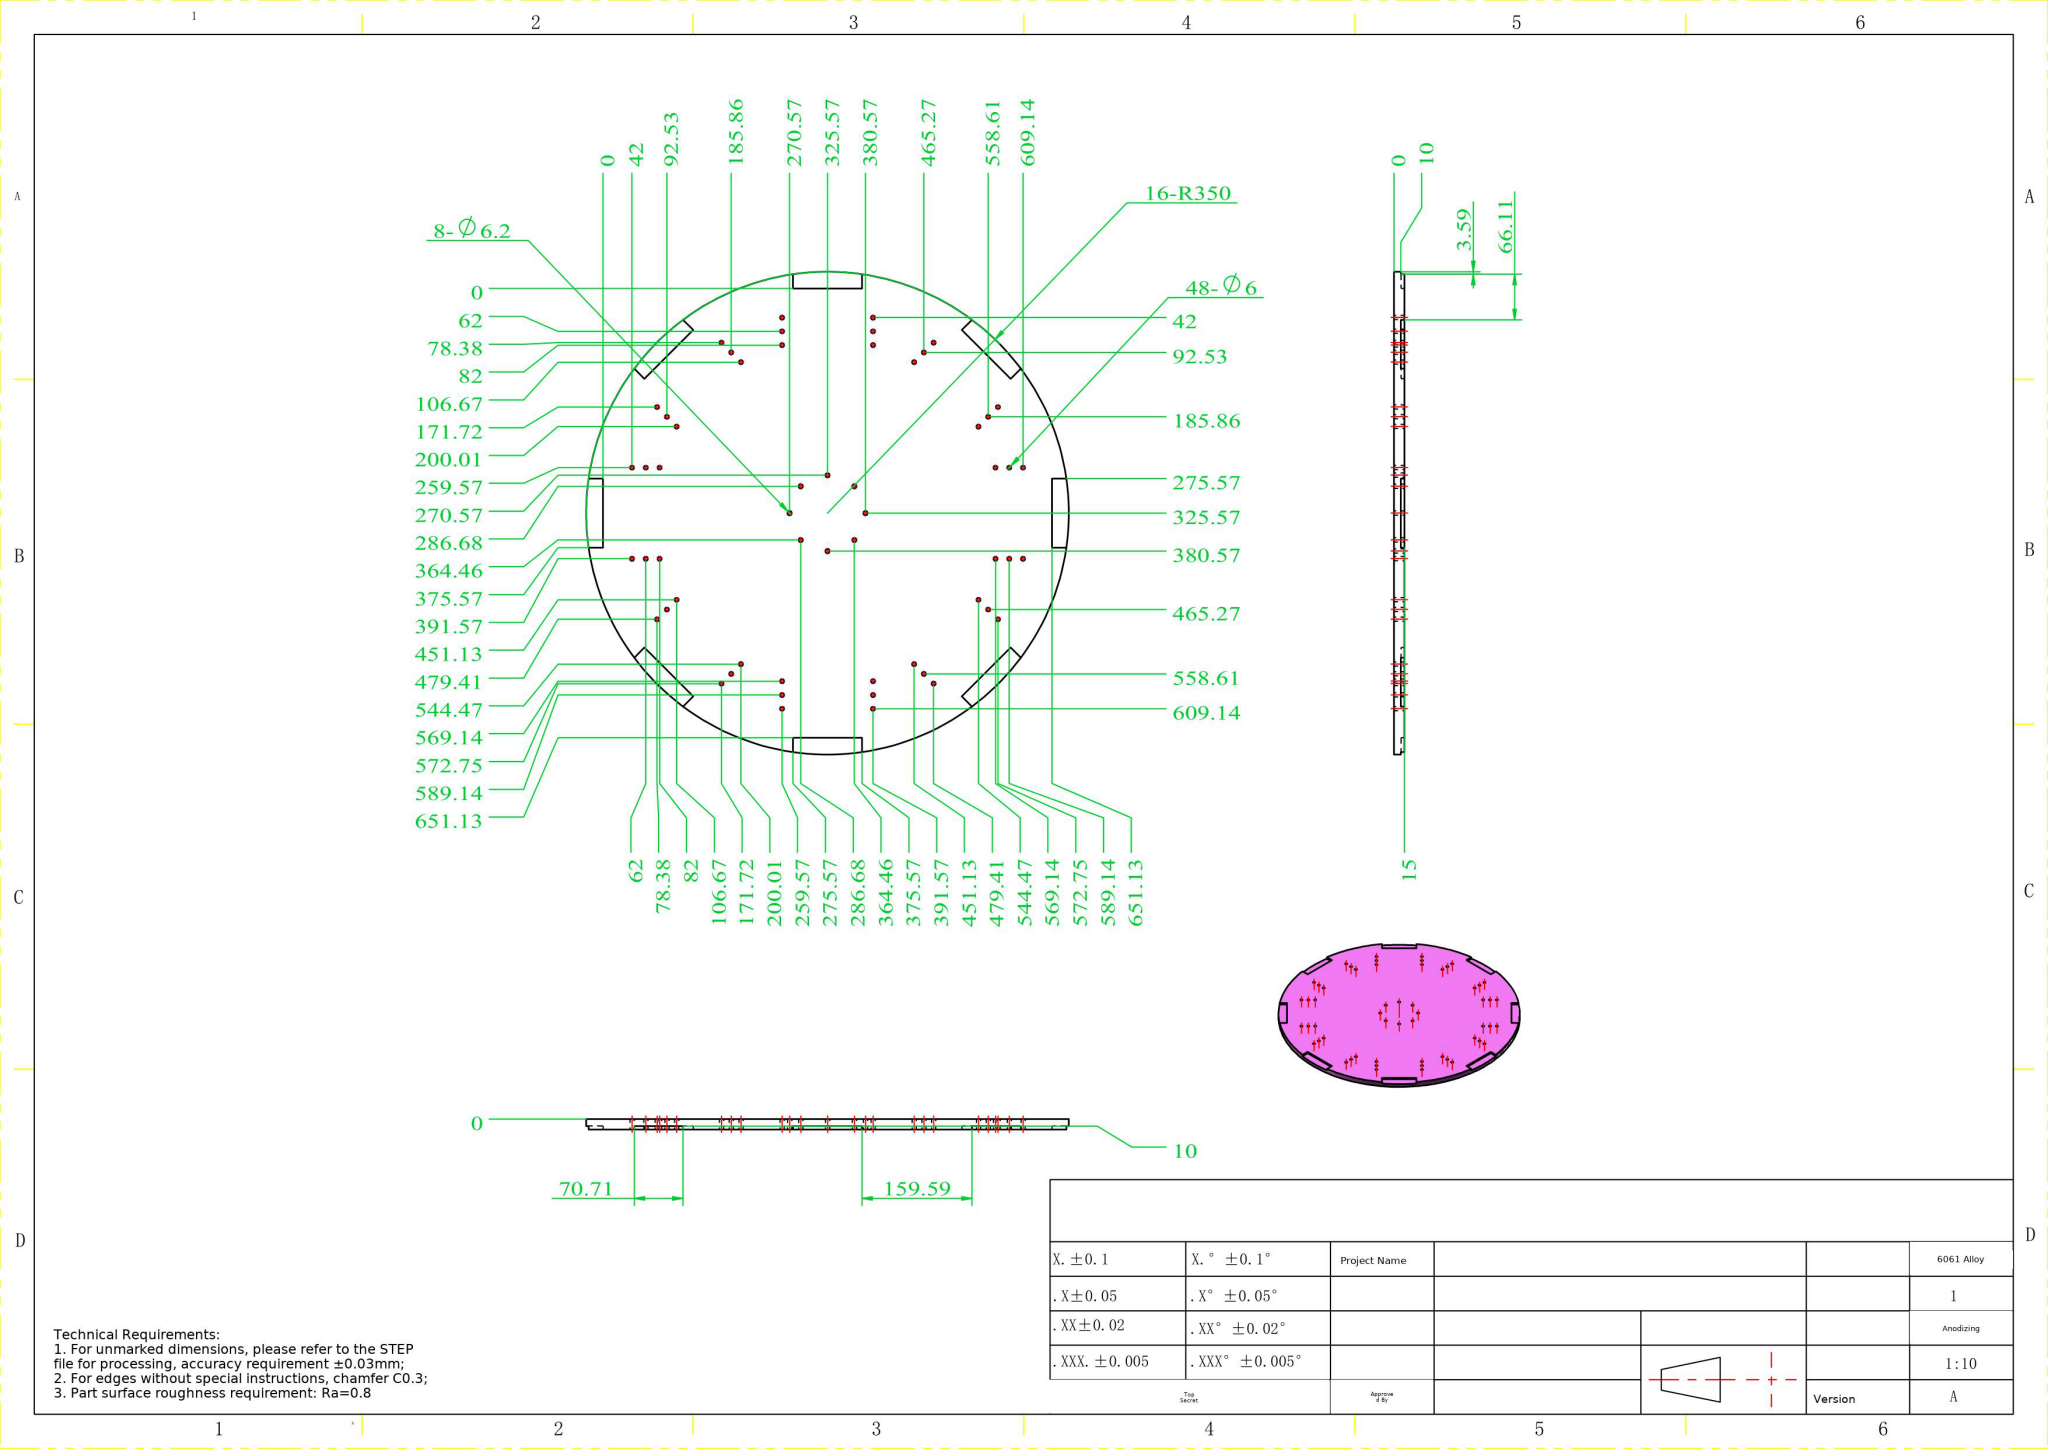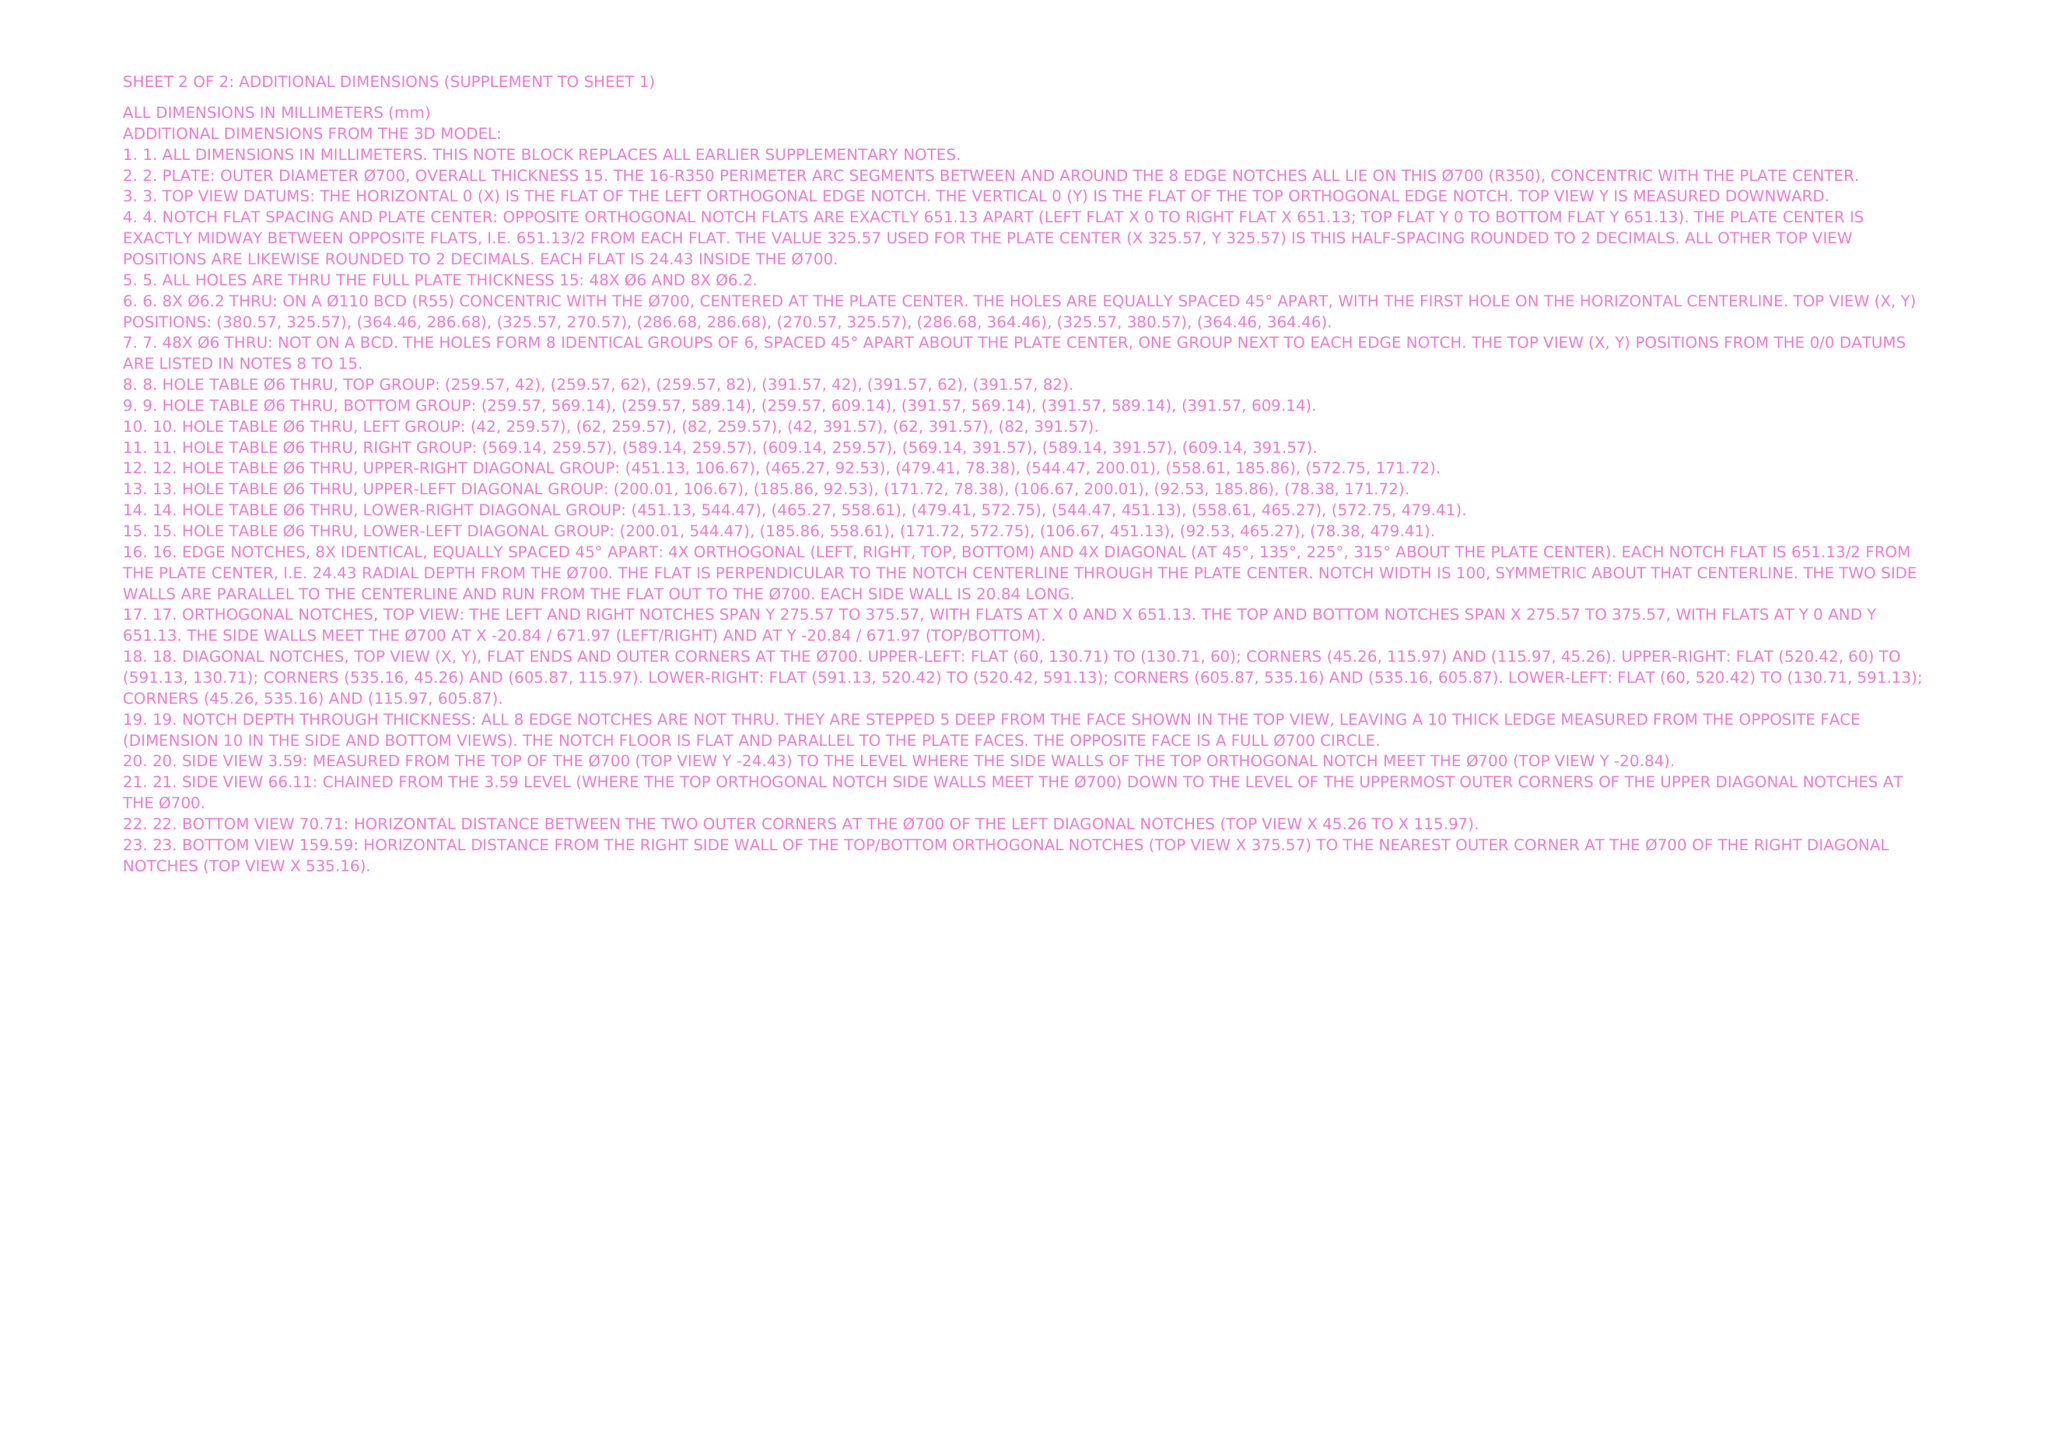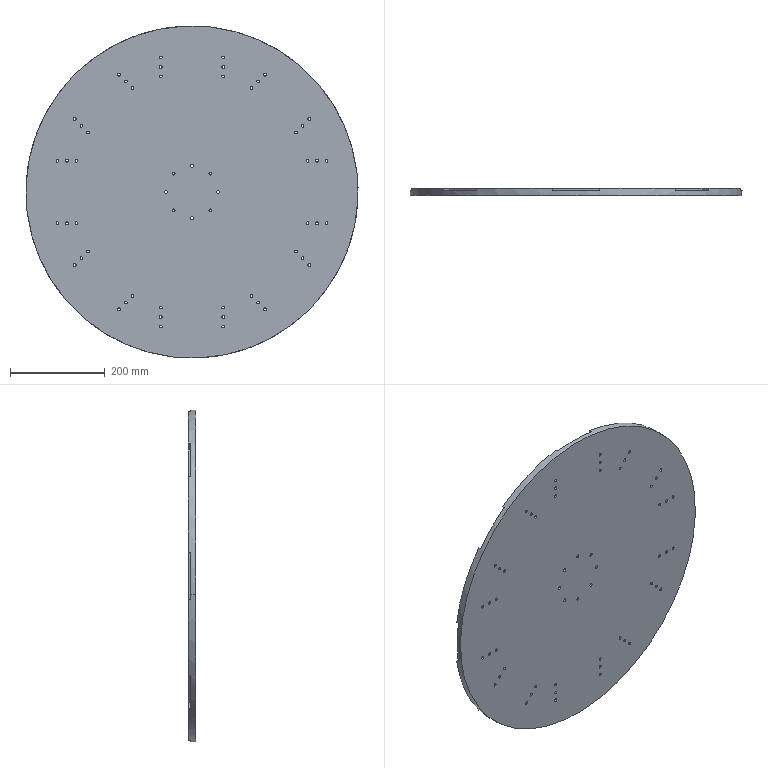Part | NX | mm | 1 solid | 148 faces | box 700 x 15 x 700 mm | volume 5655740 mm3 | cylinder 114 | plane 34 | commonest cylinder face diameters 6 x96 6.2 x16 700 x2